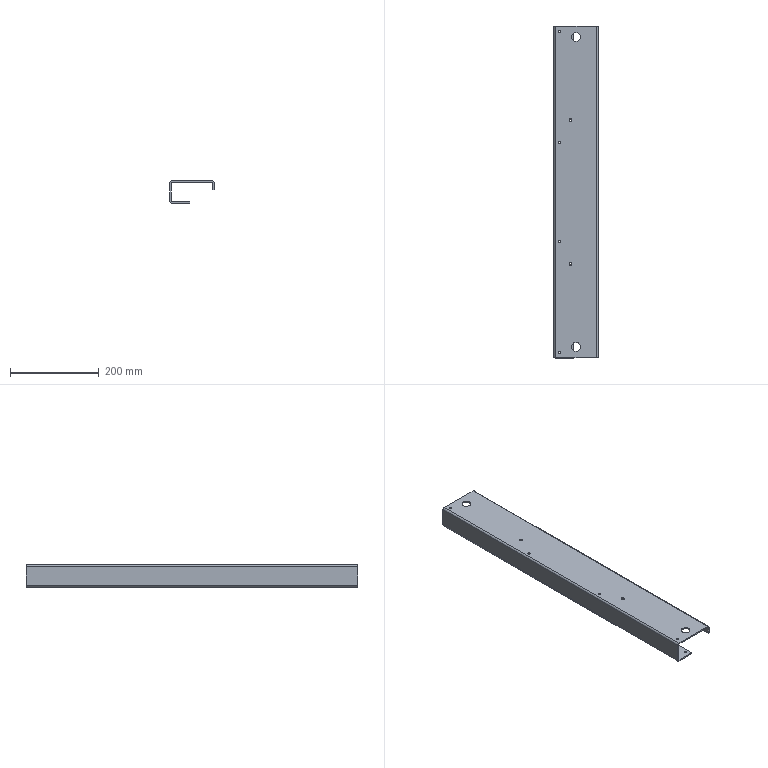Component | SolidWorks | Beam(No.15)-3 | 1 solid | 226 faces | volume 448636 mm3 | cylinder 202 | plane 24 | commonest cylinder face diameters 5 x188 6.5 x4 20 x4 8 x3 2 x3